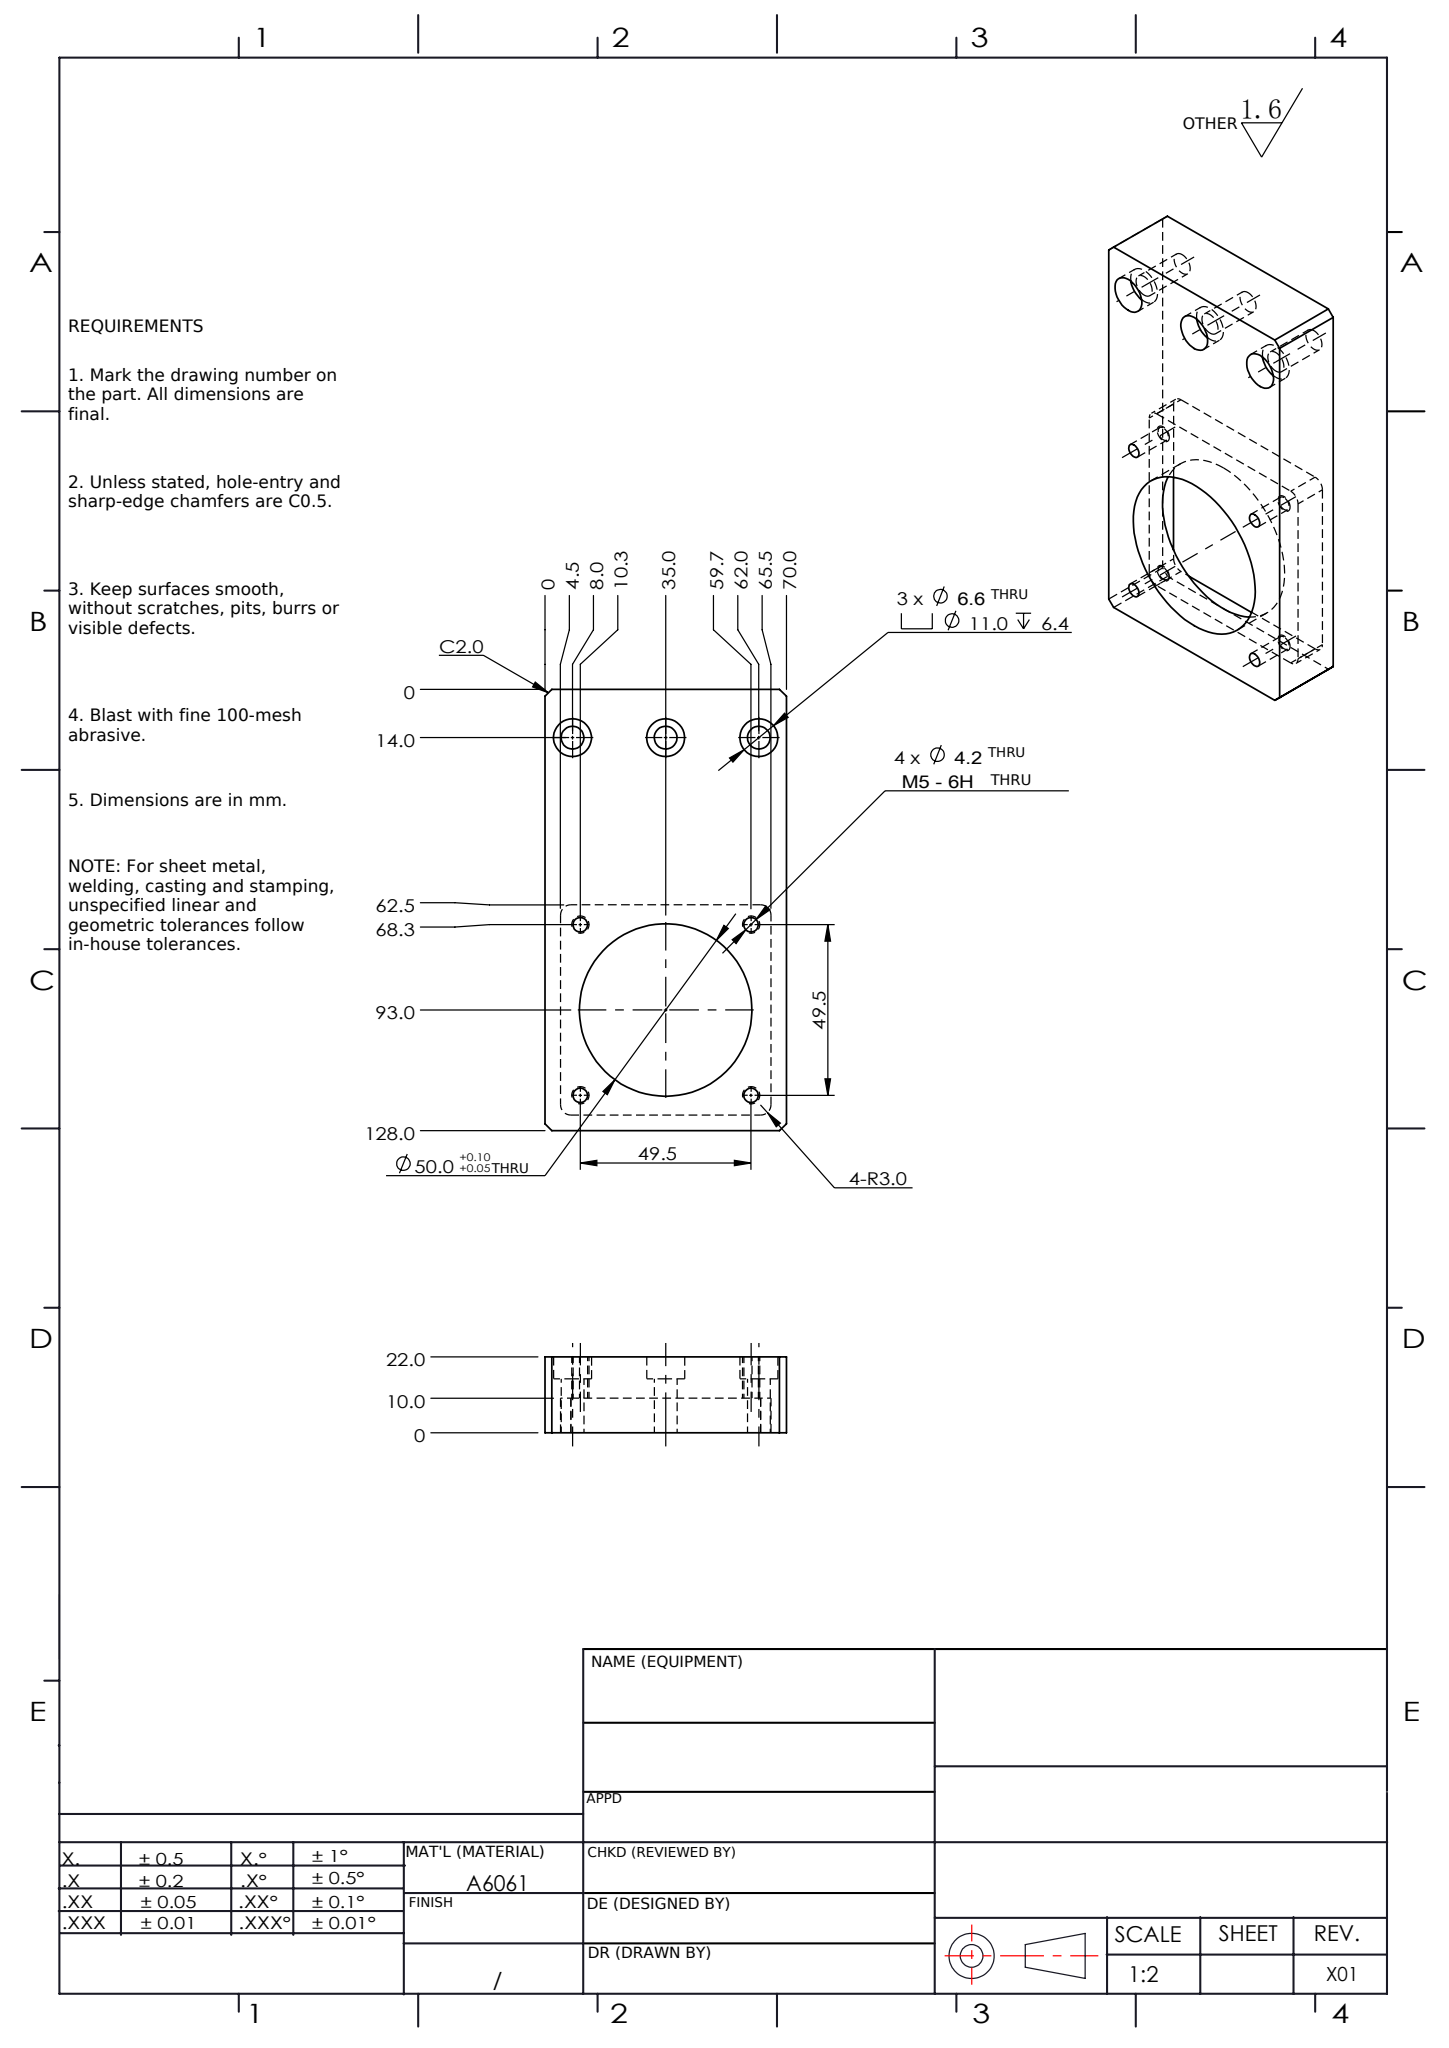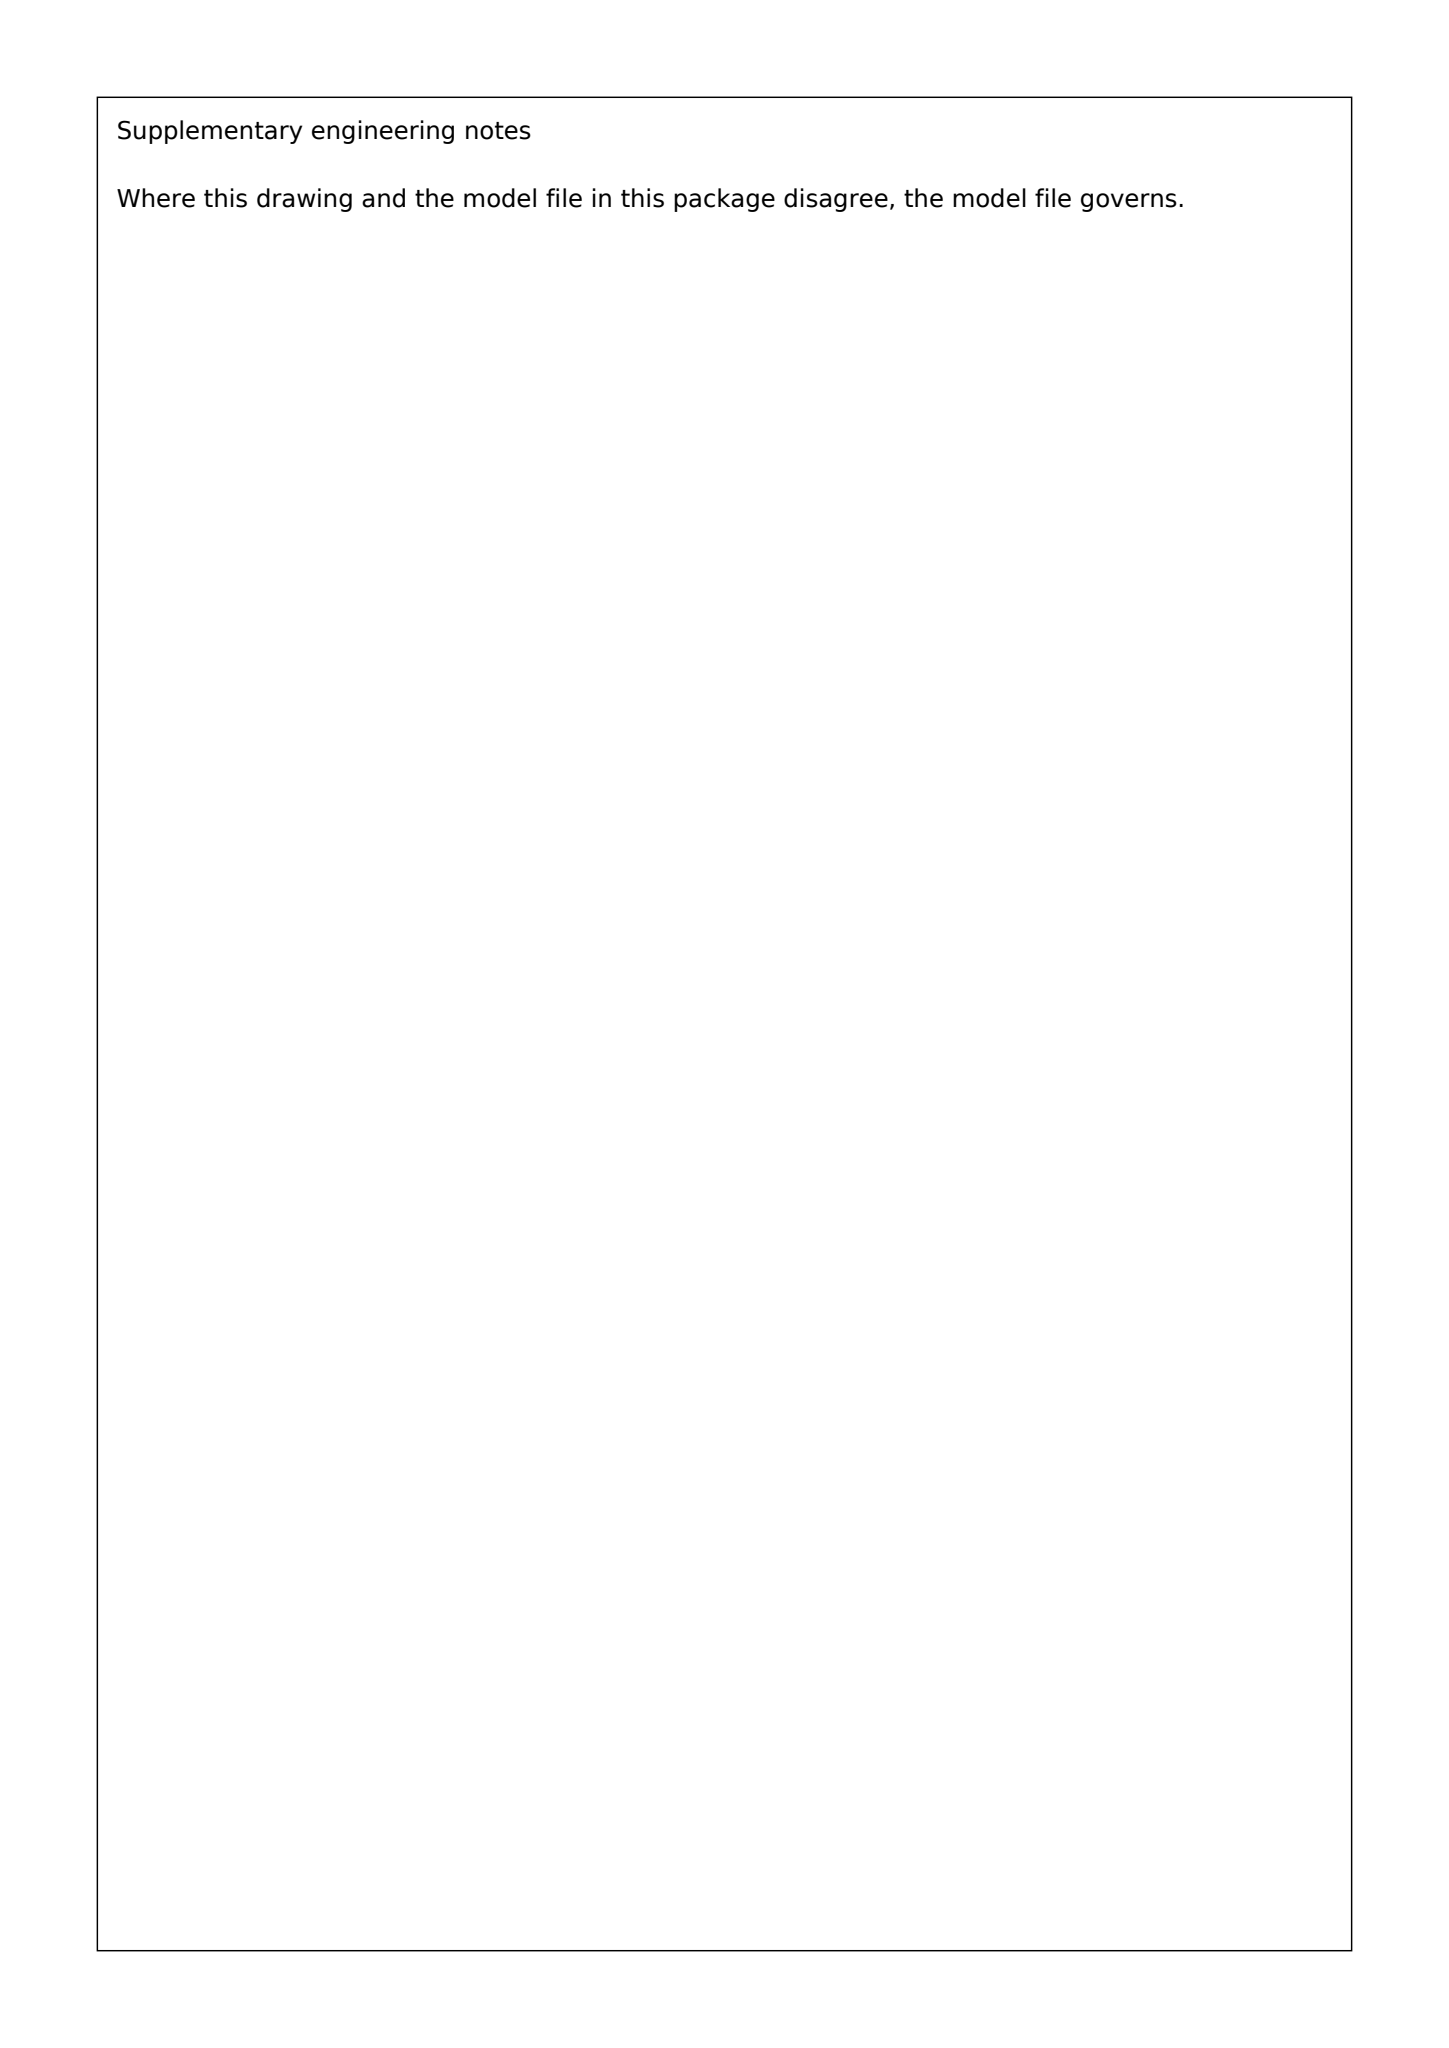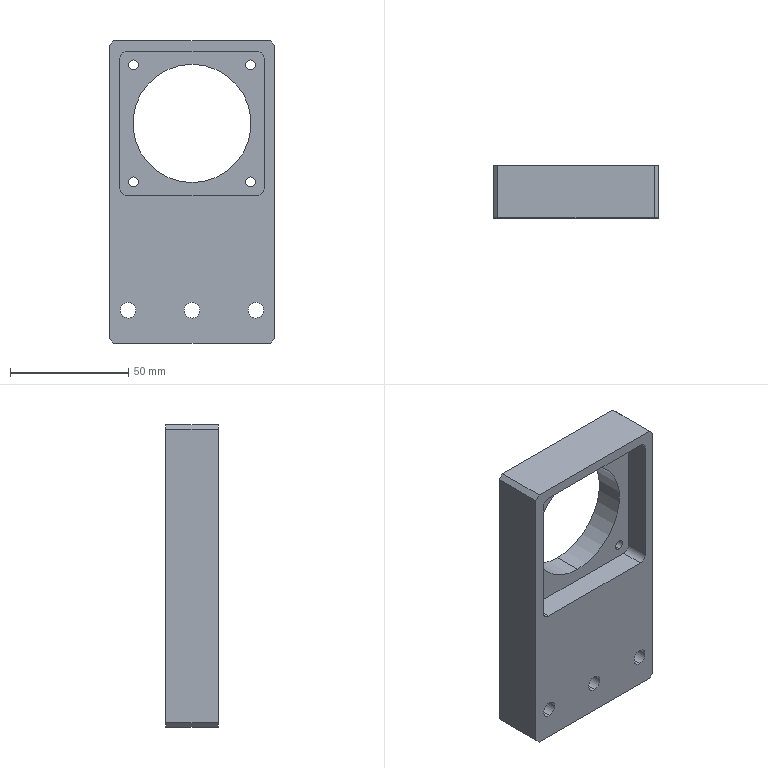Part | SolidWorks | mm | 1 solid | 44 faces | box 70 x 22 x 128 mm | volume 132159 mm3 | cylinder 26 | plane 18 | commonest cylinder face diameters 4.2 x8 11 x6 6.6 x6 6 x4 50 x2
build123d program:
from build123d import *

# Parameters (mm, degrees)
SKETCH1_W                                       = 70
SKETCH1_H                                       = 128
BOSS_EXTRUDE1_DEPTH                             = 22
SKETCH2_R                                       = 25
CUT_EXTRUDE1_DEPTH                              = 77.191
CHAMFER1_SIZE                                   = 2
SKETCH3_W                                       = 70
SKETCH3_H                                       = 8
BOSS_EXTRUDE3_DEPTH                             = 2
M6_HEX_SOCKET_HEAD_CAP_SCREW_CBORE3_D           = 6.6
M6_HEX_SOCKET_HEAD_CAP_SCREW_CBORE3_CBORE_D     = 11
M6_HEX_SOCKET_HEAD_CAP_SCREW_CBORE3_CBORE_DEPTH = 6.4
M5_TAPPED_HOLE1_D                               = 4.2
SKETCH8_W                                       = 61
SKETCH8_H                                       = 61
CUT_EXTRUDE2_DEPTH                              = 10
FILLET1_R                                       = 3
MOVE_FACE1_BY                                   = 2


with BuildPart() as part:
    # Sketch1 → Boss-Extrude1 (new body)
    with BuildSketch(Plane(origin=(0, 0, 0), x_dir=(1, 0, 0), z_dir=(0, 1, 0))):
        Rectangle(SKETCH1_W, SKETCH1_H)
    extrude(amount=BOSS_EXTRUDE1_DEPTH)

    # Sketch2 → Cut-Extrude1 (cut, through all)
    with BuildSketch(Plane(origin=(0, 22, 0), x_dir=(1, 0, 0), z_dir=(0, 1, 0))):
        with Locations(Location((0, -29, 0), (0, 0, 270))):
            Circle(SKETCH2_R)
    extrude(amount=-CUT_EXTRUDE1_DEPTH, mode=Mode.SUBTRACT)

    # Chamfer1
    chamfer1_edges = [part.edges().sort_by_distance(p)[0] for p in [
        (35, 11, 64),
        (-35, 11, 64),
        (-35, 11, -64),
        (35, 11, -64),
    ]]
    chamfer(chamfer1_edges, length=CHAMFER1_SIZE)

    # Sketch3 → Boss-Extrude3 (add)
    with BuildSketch(Plane.XZ):
        with Locations((0, -50)):
            Rectangle(SKETCH3_W, SKETCH3_H)
    extrude(amount=BOSS_EXTRUDE3_DEPTH)

    # M6 Hex Socket Head Cap Screw CBORE3 (through all)
    with Locations(Plane(origin=(0, 22, 0), x_dir=(1, 0, 0), z_dir=(0, 1, 0))):
        with Locations((-27, 50), (0, 50), (27, 50)):
            CounterBoreHole(M6_HEX_SOCKET_HEAD_CAP_SCREW_CBORE3_D / 2, M6_HEX_SOCKET_HEAD_CAP_SCREW_CBORE3_CBORE_D / 2, M6_HEX_SOCKET_HEAD_CAP_SCREW_CBORE3_CBORE_DEPTH)

    # M5 Tapped Hole1 (through all)
    with Locations(Plane(origin=(0, 0, 0), x_dir=(-1, 0, 0), z_dir=(0, -1, 0))):
        with Locations((24.749, -4.251), (24.749, -53.749), (-24.749, -53.749), (-24.749, -4.251)):
            Hole(M5_TAPPED_HOLE1_D / 2)

    # Sketch8 → Cut-Extrude2 (cut)
    with BuildSketch(Plane.XZ):
        with Locations((0, 29)):
            Rectangle(SKETCH8_W, SKETCH8_H)
    extrude(amount=-CUT_EXTRUDE2_DEPTH, mode=Mode.SUBTRACT)

    # Fillet1
    fillet1_edges = [part.edges().sort_by_distance(p)[0] for p in [
        (30.5, 5, 59.5),
        (30.5, 5, -1.5),
        (-30.5, 5, -1.5),
        (-30.5, 5, 59.5),
    ]]
    fillet(fillet1_edges, radius=FILLET1_R)

    # Move Face1: a face moved inward by 2.0
    extrude(part.faces().sort_by_distance((17.5, -2, -50))[0], amount=MOVE_FACE1_BY, dir=(0, 1, 0), mode=Mode.SUBTRACT)


solid = part.part